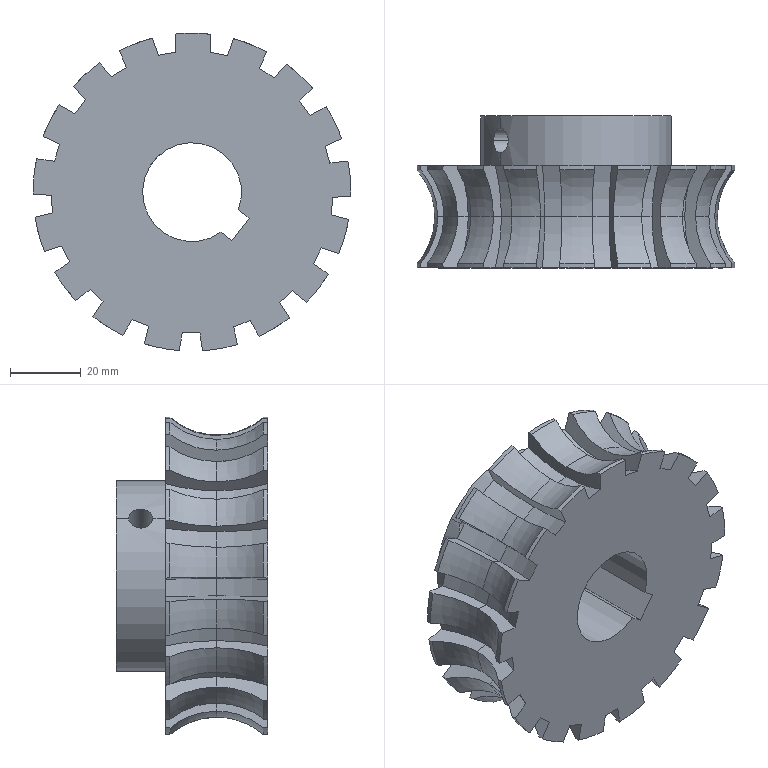Component | SolidWorks | 18-1 | 1 solid | 166 faces | volume 151907 mm3 | cylinder 73 | cone 51 | torus 36 | plane 6 | commonest cylinder face diameters 66.641 x34 90 x34 6.8 x2 54 x2 28 x1